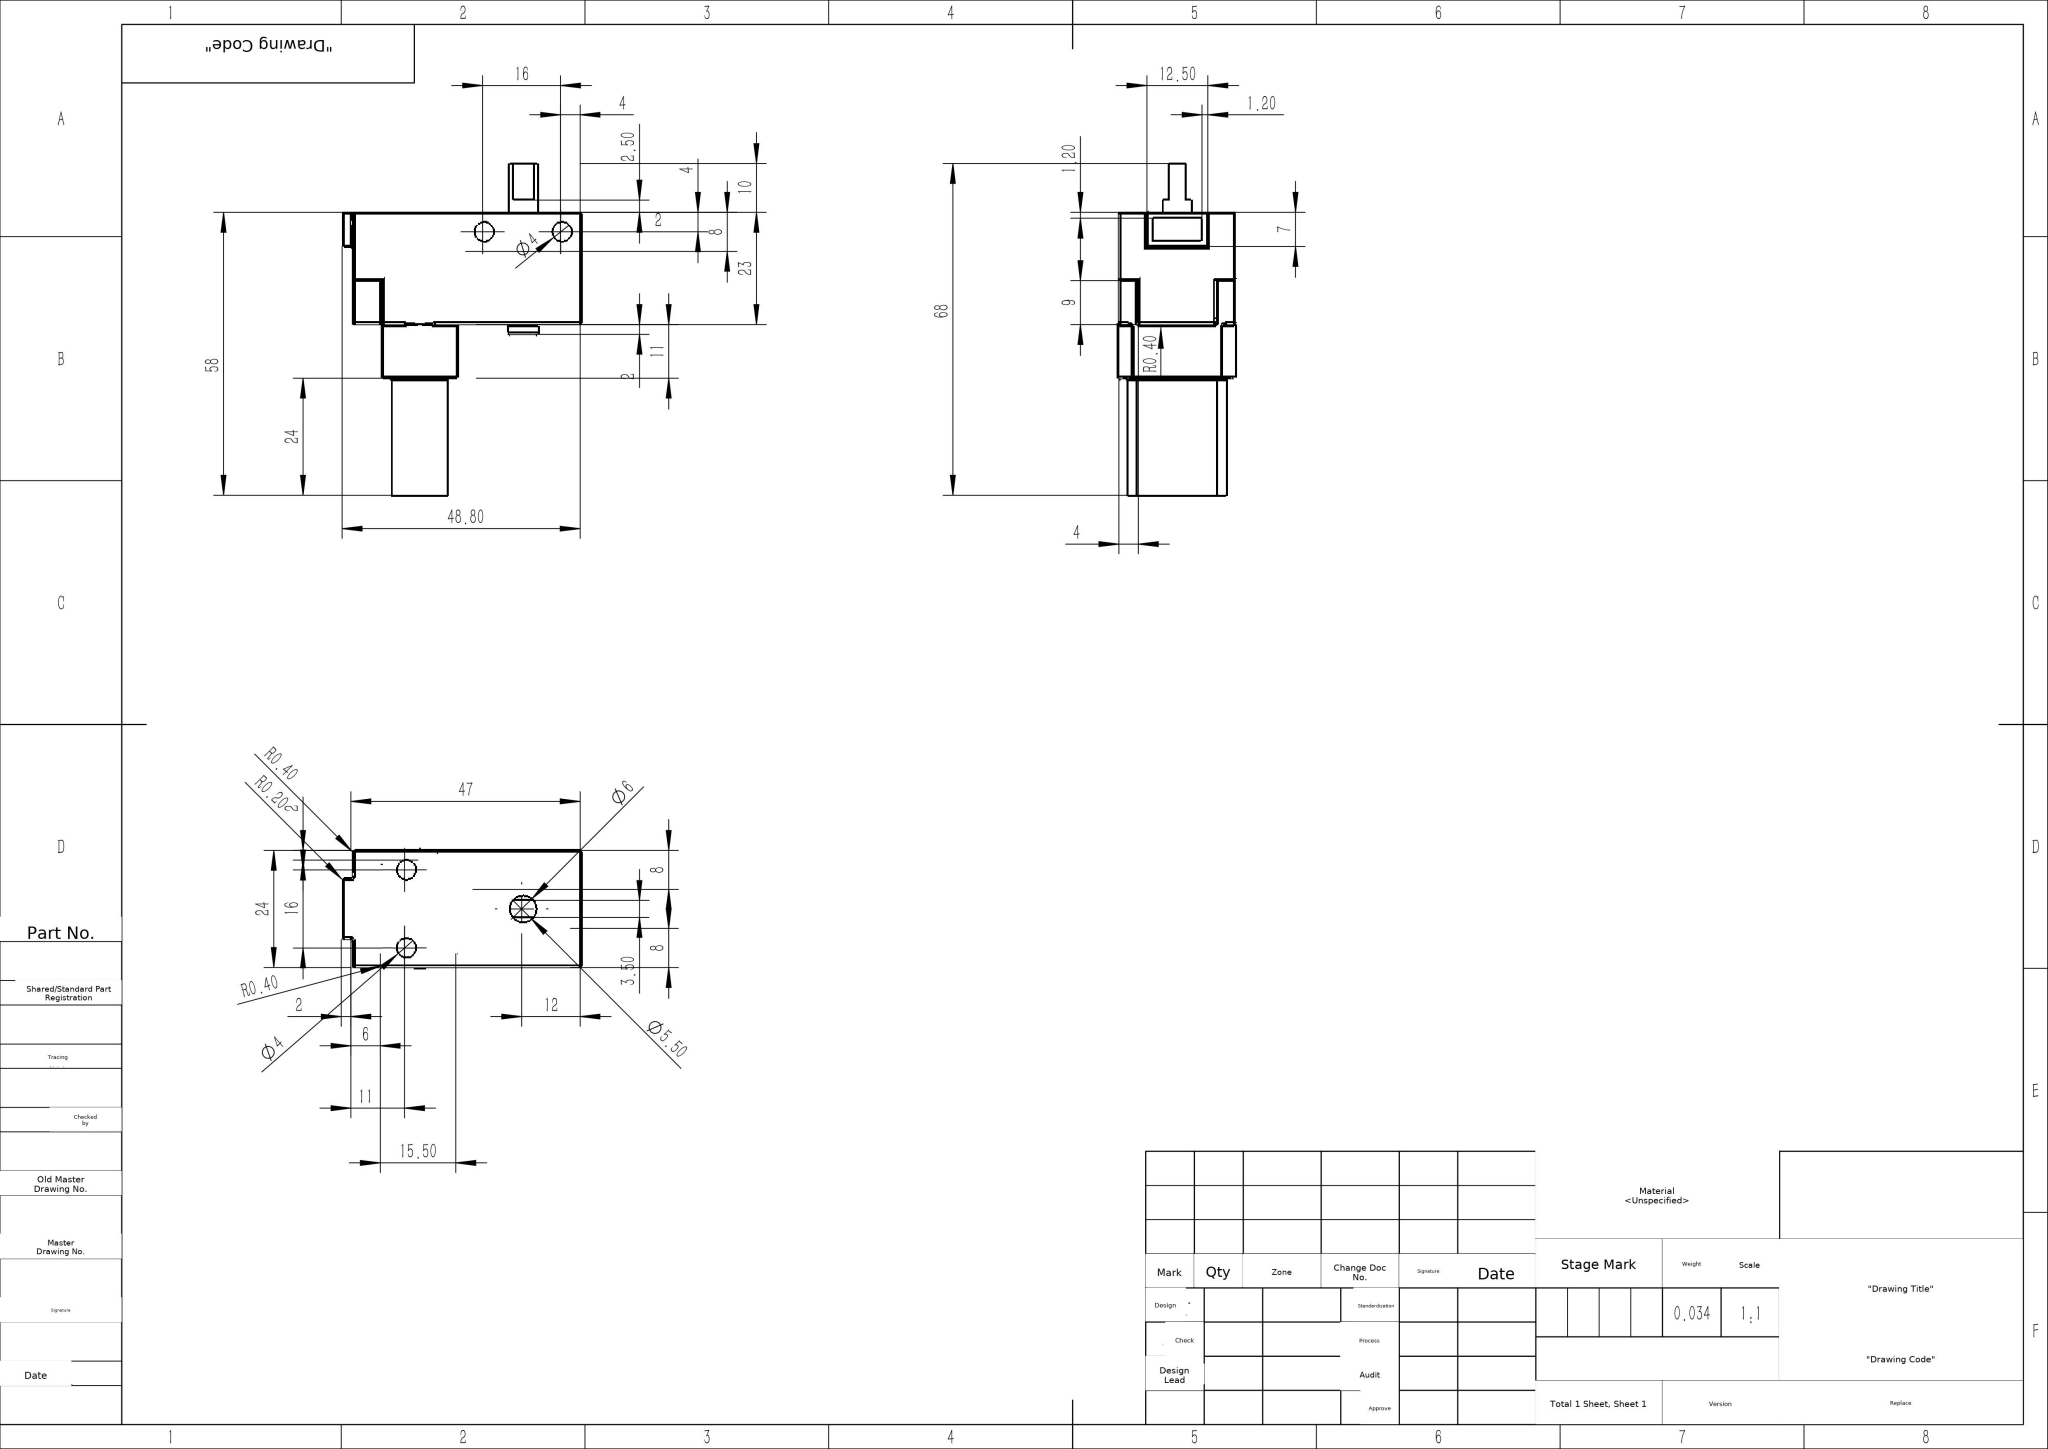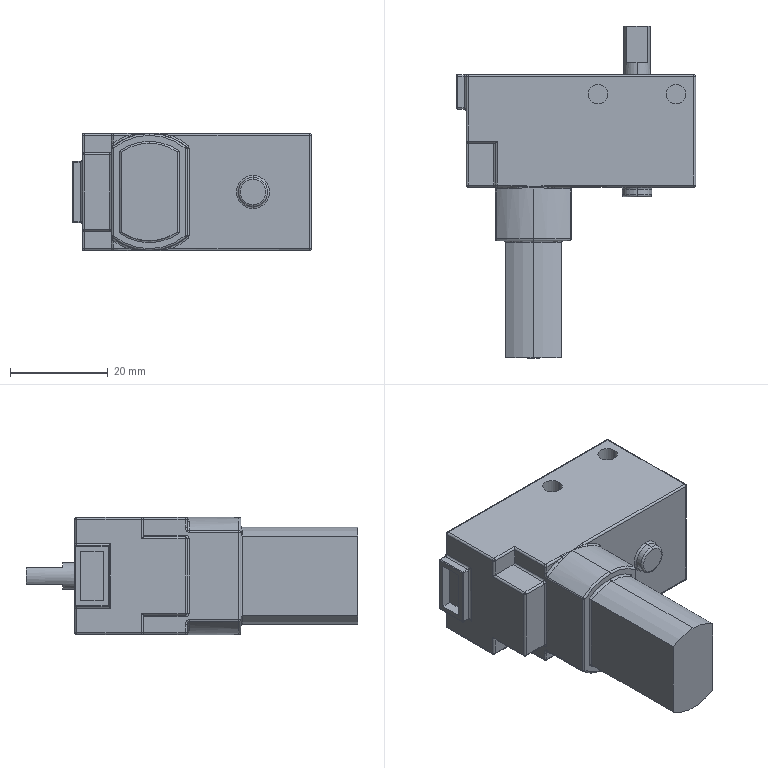Part | SolidWorks | mm | 1 solid | 168 faces | box 49 x 68 x 24 mm | volume 34215 mm3 | cylinder 72 | plane 40 | torus 22 | sphere 18 | spline 16 | commonest cylinder face diameters 0.8 x44 4 x12 0.4 x6 20 x3 24 x3 6 x2 5.5 x2